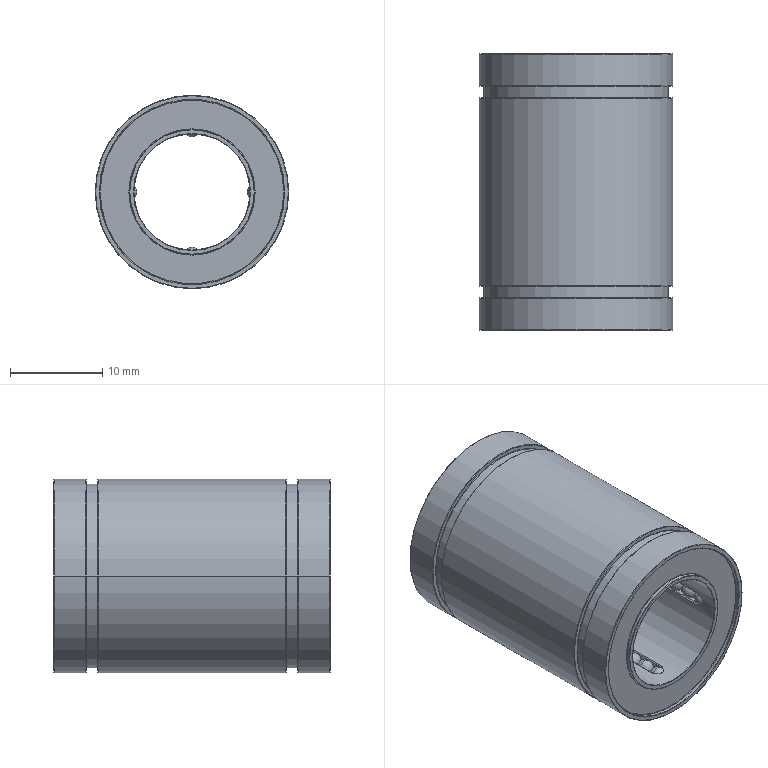Component | SolidWorks | JL001-05-03-1_LM12UU-1 | 1 solid | 328 faces | volume 6353 mm3 | cylinder 134 | sphere 112 | torus 56 | spline 16 | plane 10 | commonest cylinder face diameters 1.794 x104 0.2 x10 20 x8 21 x6 13.6 x4 12.6 x2